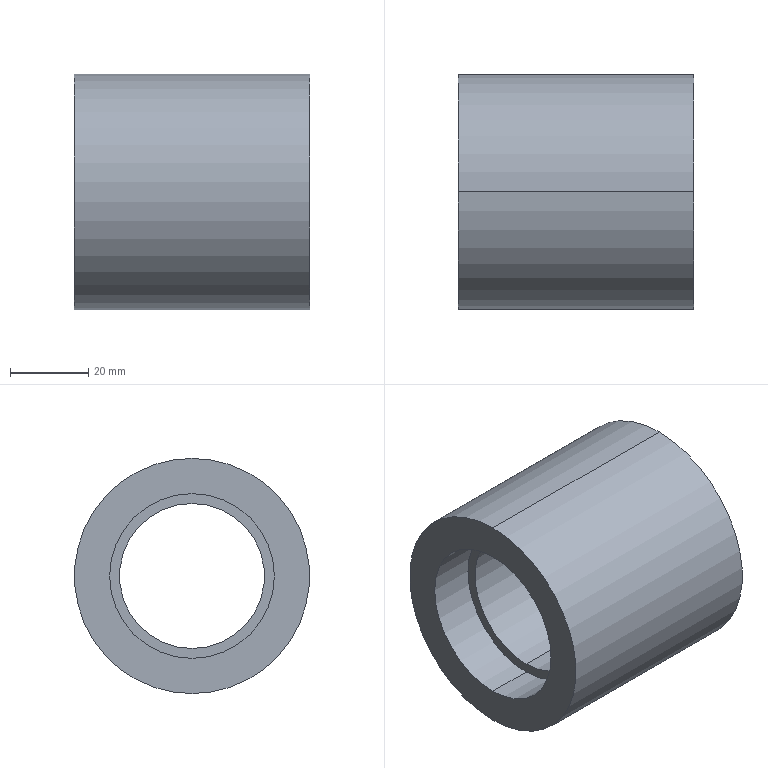Component | SolidWorks | J-TRD899MINI-2213-05PressingWheel-1 | 1 solid | 12 faces | box 60 x 60 x 60 mm | volume 97688 mm3 | cylinder 8 | plane 4 | commonest cylinder face diameters 42 x4 60 x2 37 x2 | material Urethane
build123d program:
from build123d import *


with BuildPart() as part:
    # Sketch1 → Revolve1 (revolve)
    with BuildSketch(Plane(origin=(0, 0, 0), x_dir=(0, 0, -1), z_dir=(1, 0, 0)), mode=Mode.PRIVATE) as revolve1_sk:
        Polygon((12, 21), (12, 18.5), (48, 18.5), (48, 21), (60, 21), (60, 30), (0, 30), (0, 21), align=None)
    revolve(revolve1_sk.sketch.rotate(Axis((0, 0, 0), (0, 0, -1)), 90), axis=Axis((0, 0, 0), (0, 0, -1)))


solid = part.part

# Placed as in the assembly
solid = solid.moved(Location((-48.663, 20.996, 191.6), (0, 90, 0)))
STEP:
#1=COLOUR_RGB('',0.7922,0.8196,0.9333);
#2=FILL_AREA_STYLE_COLOUR('',#1);
#3=FILL_AREA_STYLE('',(#2));
#4=SURFACE_STYLE_FILL_AREA(#3);
#5=SURFACE_SIDE_STYLE('',(#4));
#6=SURFACE_STYLE_USAGE(.BOTH.,#5);
#7=PRESENTATION_STYLE_ASSIGNMENT((#6));
#8=CARTESIAN_POINT('',(-1.916,0.8266,8.724));
#9=VERTEX_POINT('',#8);
#10=CARTESIAN_POINT('',(-1.916,0.8266,6.362));
#11=VERTEX_POINT('',#10);
#12=CARTESIAN_POINT('',(-1.916,0.8266,7.543));
#13=DIRECTION('',(-1.,0.,0.));
#14=DIRECTION('',(0.,0.,1.));
#15=AXIS2_PLACEMENT_3D('',#12,#13,#14);
#16=CIRCLE('',#15,1.181);
#17=EDGE_CURVE('',#9,#11,#16,.T.);
#18=ORIENTED_EDGE('',*,*,#17,.T.);
#19=CARTESIAN_POINT('',(-4.278,0.8266,6.362));
#20=VERTEX_POINT('',#19);
#21=CARTESIAN_POINT('',(-4.278,0.8266,6.362));
#22=DIRECTION('',(-1.,0.,0.));
#23=VECTOR('',#22,39.37);
#24=LINE('',#21,#23);
#25=EDGE_CURVE('',#11,#20,#24,.T.);
#26=ORIENTED_EDGE('',*,*,#25,.T.);
#27=CARTESIAN_POINT('',(-4.278,0.8266,8.724));
#28=VERTEX_POINT('',#27);
#29=CARTESIAN_POINT('',(-4.278,0.8266,7.543));
#30=DIRECTION('',(-1.,0.,0.));
#31=DIRECTION('',(0.,0.,1.));
#32=AXIS2_PLACEMENT_3D('',#29,#30,#31);
#33=CIRCLE('',#32,1.181);
#34=EDGE_CURVE('',#28,#20,#33,.T.);
#35=ORIENTED_EDGE('',*,*,#34,.F.);
#36=CARTESIAN_POINT('',(-4.278,0.8266,8.724));
#37=DIRECTION('',(-1.,0.,0.));
#38=VECTOR('',#37,39.37);
#39=LINE('',#36,#38);
#40=EDGE_CURVE('',#9,#28,#39,.T.);
#41=ORIENTED_EDGE('',*,*,#40,.F.);
#42=EDGE_LOOP('',(#18,#26,#35,#41));
#43=FACE_OUTER_BOUND('',#42,.T.);
#44=CARTESIAN_POINT('',(-4.278,0.8266,7.543));
#45=DIRECTION('',(-1.,0.,0.));
#46=DIRECTION('',(0.,0.,1.));
#47=AXIS2_PLACEMENT_3D('',#44,#45,#46);
#48=CYLINDRICAL_SURFACE('',#47,1.181);
#49=ADVANCED_FACE('',(#43),#48,.T.);
#50=CARTESIAN_POINT('',(-1.916,0.8266,6.717));
#51=VERTEX_POINT('',#50);
#52=CARTESIAN_POINT('',(-1.916,0.8266,8.37));
#53=VERTEX_POINT('',#52);
#54=CARTESIAN_POINT('',(-1.916,0.8266,7.543));
#55=DIRECTION('',(-1.,0.,0.));
#56=DIRECTION('',(0.,0.,1.));
#57=AXIS2_PLACEMENT_3D('',#54,#55,#56);
#58=CIRCLE('',#57,0.8268);
#59=EDGE_CURVE('',#51,#53,#58,.T.);
#60=ORIENTED_EDGE('',*,*,#59,.F.);
#61=CARTESIAN_POINT('',(-2.388,0.8266,6.717));
#62=VERTEX_POINT('',#61);
#63=CARTESIAN_POINT('',(-4.278,0.8266,6.717));
#64=DIRECTION('',(-1.,0.,0.));
#65=VECTOR('',#64,39.37);
#66=LINE('',#63,#65);
#67=EDGE_CURVE('',#51,#62,#66,.T.);
#68=ORIENTED_EDGE('',*,*,#67,.T.);
#69=CARTESIAN_POINT('',(-2.388,0.8266,8.37));
#70=VERTEX_POINT('',#69);
#71=CARTESIAN_POINT('',(-2.388,0.8266,7.543));
#72=DIRECTION('',(-1.,0.,0.));
#73=DIRECTION('',(0.,0.,1.));
#74=AXIS2_PLACEMENT_3D('',#71,#72,#73);
#75=CIRCLE('',#74,0.8268);
#76=EDGE_CURVE('',#62,#70,#75,.T.);
#77=ORIENTED_EDGE('',*,*,#76,.T.);
#78=CARTESIAN_POINT('',(-4.278,0.8266,8.37));
#79=DIRECTION('',(-1.,0.,0.));
#80=VECTOR('',#79,39.37);
#81=LINE('',#78,#80);
#82=EDGE_CURVE('',#53,#70,#81,.T.);
#83=ORIENTED_EDGE('',*,*,#82,.F.);
#84=EDGE_LOOP('',(#60,#68,#77,#83));
#85=FACE_OUTER_BOUND('',#84,.T.);
#86=CARTESIAN_POINT('',(-4.278,0.8266,7.543));
#87=DIRECTION('',(-1.,0.,0.));
#88=DIRECTION('',(0.,0.,1.));
#89=AXIS2_PLACEMENT_3D('',#86,#87,#88);
#90=CYLINDRICAL_SURFACE('',#89,0.8268);
#91=ADVANCED_FACE('',(#85),#90,.F.);
#92=CARTESIAN_POINT('',(-2.388,0.8266,6.815));
#93=VERTEX_POINT('',#92);
#94=CARTESIAN_POINT('',(-2.388,0.8266,8.272));
#95=VERTEX_POINT('',#94);
#96=CARTESIAN_POINT('',(-2.388,0.8266,7.543));
#97=DIRECTION('',(-1.,0.,0.));
#98=DIRECTION('',(0.,0.,1.));
#99=AXIS2_PLACEMENT_3D('',#96,#97,#98);
#100=CIRCLE('',#99,0.7283);
#101=EDGE_CURVE('',#93,#95,#100,.T.);
#102=ORIENTED_EDGE('',*,*,#101,.F.);
#103=CARTESIAN_POINT('',(-3.806,0.8266,6.815));
#104=VERTEX_POINT('',#103);
#105=CARTESIAN_POINT('',(-4.278,0.8266,6.815));
#106=DIRECTION('',(-1.,0.,0.));
#107=VECTOR('',#106,39.37);
#108=LINE('',#105,#107);
#109=EDGE_CURVE('',#93,#104,#108,.T.);
#110=ORIENTED_EDGE('',*,*,#109,.T.);
#111=CARTESIAN_POINT('',(-3.806,0.8266,8.272));
#112=VERTEX_POINT('',#111);
#113=CARTESIAN_POINT('',(-3.806,0.8266,7.543));
#114=DIRECTION('',(-1.,0.,0.));
#115=DIRECTION('',(0.,0.,1.));
#116=AXIS2_PLACEMENT_3D('',#113,#114,#115);
#117=CIRCLE('',#116,0.7283);
#118=EDGE_CURVE('',#104,#112,#117,.T.);
#119=ORIENTED_EDGE('',*,*,#118,.T.);
#120=CARTESIAN_POINT('',(-4.278,0.8266,8.272));
#121=DIRECTION('',(-1.,0.,0.));
#122=VECTOR('',#121,39.37);
#123=LINE('',#120,#122);
#124=EDGE_CURVE('',#95,#112,#123,.T.);
#125=ORIENTED_EDGE('',*,*,#124,.F.);
#126=EDGE_LOOP('',(#102,#110,#119,#125));
#127=FACE_OUTER_BOUND('',#126,.T.);
#128=CARTESIAN_POINT('',(-4.278,0.8266,7.543));
#129=DIRECTION('',(-1.,0.,0.));
#130=DIRECTION('',(0.,0.,1.));
#131=AXIS2_PLACEMENT_3D('',#128,#129,#130);
#132=CYLINDRICAL_SURFACE('',#131,0.7283);
#133=ADVANCED_FACE('',(#127),#132,.F.);
#134=CARTESIAN_POINT('',(-3.806,0.8266,6.717));
#135=VERTEX_POINT('',#134);
#136=CARTESIAN_POINT('',(-3.806,0.8266,8.37));
#137=VERTEX_POINT('',#136);
#138=CARTESIAN_POINT('',(-3.806,0.8266,7.543));
#139=DIRECTION('',(-1.,0.,0.));
#140=DIRECTION('',(0.,0.,1.));
#141=AXIS2_PLACEMENT_3D('',#138,#139,#140);
#142=CIRCLE('',#141,0.8268);
#143=EDGE_CURVE('',#135,#137,#142,.T.);
#144=ORIENTED_EDGE('',*,*,#143,.F.);
#145=CARTESIAN_POINT('',(-4.278,0.8266,6.717));
#146=VERTEX_POINT('',#145);
#147=CARTESIAN_POINT('',(-4.278,0.8266,6.717));
#148=DIRECTION('',(-1.,0.,0.));
#149=VECTOR('',#148,39.37);
#150=LINE('',#147,#149);
#151=EDGE_CURVE('',#135,#146,#150,.T.);
#152=ORIENTED_EDGE('',*,*,#151,.T.);
#153=CARTESIAN_POINT('',(-4.278,0.8266,8.37));
#154=VERTEX_POINT('',#153);
#155=CARTESIAN_POINT('',(-4.278,0.8266,7.543));
#156=DIRECTION('',(-1.,0.,0.));
#157=DIRECTION('',(0.,0.,1.));
#158=AXIS2_PLACEMENT_3D('',#155,#156,#157);
#159=CIRCLE('',#158,0.8268);
#160=EDGE_CURVE('',#146,#154,#159,.T.);
#161=ORIENTED_EDGE('',*,*,#160,.T.);
#162=CARTESIAN_POINT('',(-4.278,0.8266,8.37));
#163=DIRECTION('',(-1.,0.,0.));
#164=VECTOR('',#163,39.37);
#165=LINE('',#162,#164);
#166=EDGE_CURVE('',#137,#154,#165,.T.);
#167=ORIENTED_EDGE('',*,*,#166,.F.);
#168=EDGE_LOOP('',(#144,#152,#161,#167));
#169=FACE_OUTER_BOUND('',#168,.T.);
#170=CARTESIAN_POINT('',(-4.278,0.8266,7.543));
#171=DIRECTION('',(-1.,0.,0.));
#172=DIRECTION('',(0.,0.,1.));
#173=AXIS2_PLACEMENT_3D('',#170,#171,#172);
#174=CYLINDRICAL_SURFACE('',#173,0.8268);
#175=ADVANCED_FACE('',(#169),#174,.F.);
#176=CARTESIAN_POINT('',(-4.278,0.8266,7.543));
#177=DIRECTION('',(-1.,0.,0.));
#178=DIRECTION('',(0.,0.,1.));
#179=AXIS2_PLACEMENT_3D('',#176,#177,#178);
#180=CIRCLE('',#179,0.8268);
#181=EDGE_CURVE('',#154,#146,#180,.T.);
#182=ORIENTED_EDGE('',*,*,#181,.F.);
#183=ORIENTED_EDGE('',*,*,#160,.F.);
#184=EDGE_LOOP('',(#182,#183));
#185=FACE_BOUND('',#184,.T.);
#186=ORIENTED_EDGE('',*,*,#34,.T.);
#187=CARTESIAN_POINT('',(-4.278,0.8266,7.543));
#188=DIRECTION('',(-1.,0.,0.));
#189=DIRECTION('',(0.,0.,1.));
#190=AXIS2_PLACEMENT_3D('',#187,#188,#189);
#191=CIRCLE('',#190,1.181);
#192=EDGE_CURVE('',#20,#28,#191,.T.);
#193=ORIENTED_EDGE('',*,*,#192,.T.);
#194=EDGE_LOOP('',(#186,#193));
#195=FACE_OUTER_BOUND('',#194,.T.);
#196=CARTESIAN_POINT('',(-4.278,2.008,7.543));
#197=DIRECTION('',(1.,0.,0.));
#198=DIRECTION('',(0.,0.,-1.));
#199=AXIS2_PLACEMENT_3D('',#196,#197,#198);
#200=PLANE('',#199);
#201=ADVANCED_FACE('',(#185,#195),#200,.F.);
#202=ORIENTED_EDGE('',*,*,#151,.F.);
#203=CARTESIAN_POINT('',(-3.806,0.8266,7.543));
#204=DIRECTION('',(-1.,0.,0.));
#205=DIRECTION('',(0.,0.,1.));
#206=AXIS2_PLACEMENT_3D('',#203,#204,#205);
#207=CIRCLE('',#206,0.8268);
#208=EDGE_CURVE('',#137,#135,#207,.T.);
#209=ORIENTED_EDGE('',*,*,#208,.F.);
#210=ORIENTED_EDGE('',*,*,#166,.T.);
#211=ORIENTED_EDGE('',*,*,#181,.T.);
#212=EDGE_LOOP('',(#202,#209,#210,#211));
#213=FACE_OUTER_BOUND('',#212,.T.);
#214=CARTESIAN_POINT('',(-4.278,0.8266,7.543));
#215=DIRECTION('',(-1.,0.,0.));
#216=DIRECTION('',(0.,0.,1.));
#217=AXIS2_PLACEMENT_3D('',#214,#215,#216);
#218=CYLINDRICAL_SURFACE('',#217,0.8268);
#219=ADVANCED_FACE('',(#213),#218,.F.);
#220=CARTESIAN_POINT('',(-3.806,0.8266,7.543));
#221=DIRECTION('',(-1.,0.,0.));
#222=DIRECTION('',(0.,0.,1.));
#223=AXIS2_PLACEMENT_3D('',#220,#221,#222);
#224=CIRCLE('',#223,0.7283);
#225=EDGE_CURVE('',#112,#104,#224,.T.);
#226=ORIENTED_EDGE('',*,*,#225,.F.);
#227=ORIENTED_EDGE('',*,*,#118,.F.);
#228=EDGE_LOOP('',(#226,#227));
#229=FACE_BOUND('',#228,.T.);
#230=ORIENTED_EDGE('',*,*,#208,.T.);
#231=ORIENTED_EDGE('',*,*,#143,.T.);
#232=EDGE_LOOP('',(#230,#231));
#233=FACE_OUTER_BOUND('',#232,.T.);
#234=CARTESIAN_POINT('',(-3.806,1.653,7.543));
#235=DIRECTION('',(1.,0.,0.));
#236=DIRECTION('',(0.,0.,-1.));
#237=AXIS2_PLACEMENT_3D('',#234,#235,#236);
#238=PLANE('',#237);
#239=ADVANCED_FACE('',(#229,#233),#238,.F.);
#240=ORIENTED_EDGE('',*,*,#109,.F.);
#241=CARTESIAN_POINT('',(-2.388,0.8266,7.543));
#242=DIRECTION('',(-1.,0.,0.));
#243=DIRECTION('',(0.,0.,1.));
#244=AXIS2_PLACEMENT_3D('',#241,#242,#243);
#245=CIRCLE('',#244,0.7283);
#246=EDGE_CURVE('',#95,#93,#245,.T.);
#247=ORIENTED_EDGE('',*,*,#246,.F.);
#248=ORIENTED_EDGE('',*,*,#124,.T.);
#249=ORIENTED_EDGE('',*,*,#225,.T.);
#250=EDGE_LOOP('',(#240,#247,#248,#249));
#251=FACE_OUTER_BOUND('',#250,.T.);
#252=CARTESIAN_POINT('',(-4.278,0.8266,7.543));
#253=DIRECTION('',(-1.,0.,0.));
#254=DIRECTION('',(0.,0.,1.));
#255=AXIS2_PLACEMENT_3D('',#252,#253,#254);
#256=CYLINDRICAL_SURFACE('',#255,0.7283);
#257=ADVANCED_FACE('',(#251),#256,.F.);
#258=CARTESIAN_POINT('',(-2.388,0.8266,7.543));
#259=DIRECTION('',(-1.,0.,0.));
#260=DIRECTION('',(0.,0.,1.));
#261=AXIS2_PLACEMENT_3D('',#258,#259,#260);
#262=CIRCLE('',#261,0.8268);
#263=EDGE_CURVE('',#70,#62,#262,.T.);
#264=ORIENTED_EDGE('',*,*,#263,.F.);
#265=ORIENTED_EDGE('',*,*,#76,.F.);
#266=EDGE_LOOP('',(#264,#265));
#267=FACE_OUTER_BOUND('',#266,.T.);
#268=ORIENTED_EDGE('',*,*,#246,.T.);
#269=ORIENTED_EDGE('',*,*,#101,.T.);
#270=EDGE_LOOP('',(#268,#269));
#271=FACE_BOUND('',#270,.T.);
#272=CARTESIAN_POINT('',(-2.388,1.555,7.543));
#273=DIRECTION('',(-1.,0.,0.));
#274=DIRECTION('',(0.,0.,1.));
#275=AXIS2_PLACEMENT_3D('',#272,#273,#274);
#276=PLANE('',#275);
#277=ADVANCED_FACE('',(#267,#271),#276,.F.);
#278=ORIENTED_EDGE('',*,*,#67,.F.);
#279=CARTESIAN_POINT('',(-1.916,0.8266,7.543));
#280=DIRECTION('',(-1.,0.,0.));
#281=DIRECTION('',(0.,0.,1.));
#282=AXIS2_PLACEMENT_3D('',#279,#280,#281);
#283=CIRCLE('',#282,0.8268);
#284=EDGE_CURVE('',#53,#51,#283,.T.);
#285=ORIENTED_EDGE('',*,*,#284,.F.);
#286=ORIENTED_EDGE('',*,*,#82,.T.);
#287=ORIENTED_EDGE('',*,*,#263,.T.);
#288=EDGE_LOOP('',(#278,#285,#286,#287));
#289=FACE_OUTER_BOUND('',#288,.T.);
#290=CARTESIAN_POINT('',(-4.278,0.8266,7.543));
#291=DIRECTION('',(-1.,0.,0.));
#292=DIRECTION('',(0.,0.,1.));
#293=AXIS2_PLACEMENT_3D('',#290,#291,#292);
#294=CYLINDRICAL_SURFACE('',#293,0.8268);
#295=ADVANCED_FACE('',(#289),#294,.F.);
#296=ORIENTED_EDGE('',*,*,#17,.F.);
#297=CARTESIAN_POINT('',(-1.916,0.8266,7.543));
#298=DIRECTION('',(-1.,0.,0.));
#299=DIRECTION('',(0.,0.,1.));
#300=AXIS2_PLACEMENT_3D('',#297,#298,#299);
#301=CIRCLE('',#300,1.181);
#302=EDGE_CURVE('',#11,#9,#301,.T.);
#303=ORIENTED_EDGE('',*,*,#302,.F.);
#304=EDGE_LOOP('',(#296,#303));
#305=FACE_OUTER_BOUND('',#304,.T.);
#306=ORIENTED_EDGE('',*,*,#284,.T.);
#307=ORIENTED_EDGE('',*,*,#59,.T.);
#308=EDGE_LOOP('',(#306,#307));
#309=FACE_BOUND('',#308,.T.);
#310=CARTESIAN_POINT('',(-1.916,2.008,7.543));
#311=DIRECTION('',(-1.,0.,0.));
#312=DIRECTION('',(0.,0.,1.));
#313=AXIS2_PLACEMENT_3D('',#310,#311,#312);
#314=PLANE('',#313);
#315=ADVANCED_FACE('',(#305,#309),#314,.F.);
#316=ORIENTED_EDGE('',*,*,#25,.F.);
#317=ORIENTED_EDGE('',*,*,#302,.T.);
#318=ORIENTED_EDGE('',*,*,#40,.T.);
#319=ORIENTED_EDGE('',*,*,#192,.F.);
#320=EDGE_LOOP('',(#316,#317,#318,#319));
#321=FACE_OUTER_BOUND('',#320,.T.);
#322=CARTESIAN_POINT('',(-4.278,0.8266,7.543));
#323=DIRECTION('',(-1.,0.,0.));
#324=DIRECTION('',(0.,0.,1.));
#325=AXIS2_PLACEMENT_3D('',#322,#323,#324);
#326=CYLINDRICAL_SURFACE('',#325,1.181);
#327=ADVANCED_FACE('',(#321),#326,.T.);
#328=CLOSED_SHELL('',(#49,#91,#133,#175,#201,#219,#239,#257,#277,#295,#315,#327));
#329=MANIFOLD_SOLID_BREP('',#328);
#330=STYLED_ITEM('',(#7),#329);
#331=(LENGTH_UNIT()NAMED_UNIT(*)SI_UNIT($,.METRE.));
#332=LENGTH_MEASURE_WITH_UNIT(LENGTH_MEASURE(0.0254),#331);
#333=DIMENSIONAL_EXPONENTS(1.,0.,0.,0.,0.,0.,0.);
#334=(CONVERSION_BASED_UNIT('',#332)LENGTH_UNIT()NAMED_UNIT(#333));
#335=UNCERTAINTY_MEASURE_WITH_UNIT(LENGTH_MEASURE(0.00001),#334,'','');
#336=(NAMED_UNIT(*)PLANE_ANGLE_UNIT()SI_UNIT($,.RADIAN.));
#337=(NAMED_UNIT(*)SI_UNIT($,.STERADIAN.)SOLID_ANGLE_UNIT());
#338=(GEOMETRIC_REPRESENTATION_CONTEXT(3)GLOBAL_UNCERTAINTY_ASSIGNED_CONTEXT((#335))GLOBAL_UNIT_ASSIGNED_CONTEXT((#334,#336,#337))REPRESENTATION_CONTEXT('',''));
#339=MECHANICAL_DESIGN_GEOMETRIC_PRESENTATION_REPRESENTATION('',(#330),#338);
#340=PRESENTATION_LAYER_ASSIGNMENT('','',(#330));
#341=CARTESIAN_POINT('',(0.,0.,0.));
#342=DIRECTION('',(0.,0.,1.));
#343=DIRECTION('',(1.,0.,0.));
#344=AXIS2_PLACEMENT_3D('',#341,#342,#343);
#345=(LENGTH_UNIT()NAMED_UNIT(*)SI_UNIT($,.METRE.));
#346=LENGTH_MEASURE_WITH_UNIT(LENGTH_MEASURE(0.0254),#345);
#347=DIMENSIONAL_EXPONENTS(1.,0.,0.,0.,0.,0.,0.);
#348=(CONVERSION_BASED_UNIT('',#346)LENGTH_UNIT()NAMED_UNIT(#347));
#349=UNCERTAINTY_MEASURE_WITH_UNIT(LENGTH_MEASURE(0.00001),#348,'','');
#350=(NAMED_UNIT(*)PLANE_ANGLE_UNIT()SI_UNIT($,.RADIAN.));
#351=(NAMED_UNIT(*)SI_UNIT($,.STERADIAN.)SOLID_ANGLE_UNIT());
#352=(GEOMETRIC_REPRESENTATION_CONTEXT(3)GLOBAL_UNCERTAINTY_ASSIGNED_CONTEXT((#349))GLOBAL_UNIT_ASSIGNED_CONTEXT((#348,#350,#351))REPRESENTATION_CONTEXT('',''));
#353=ADVANCED_BREP_SHAPE_REPRESENTATION('',(#329,#344),#352);